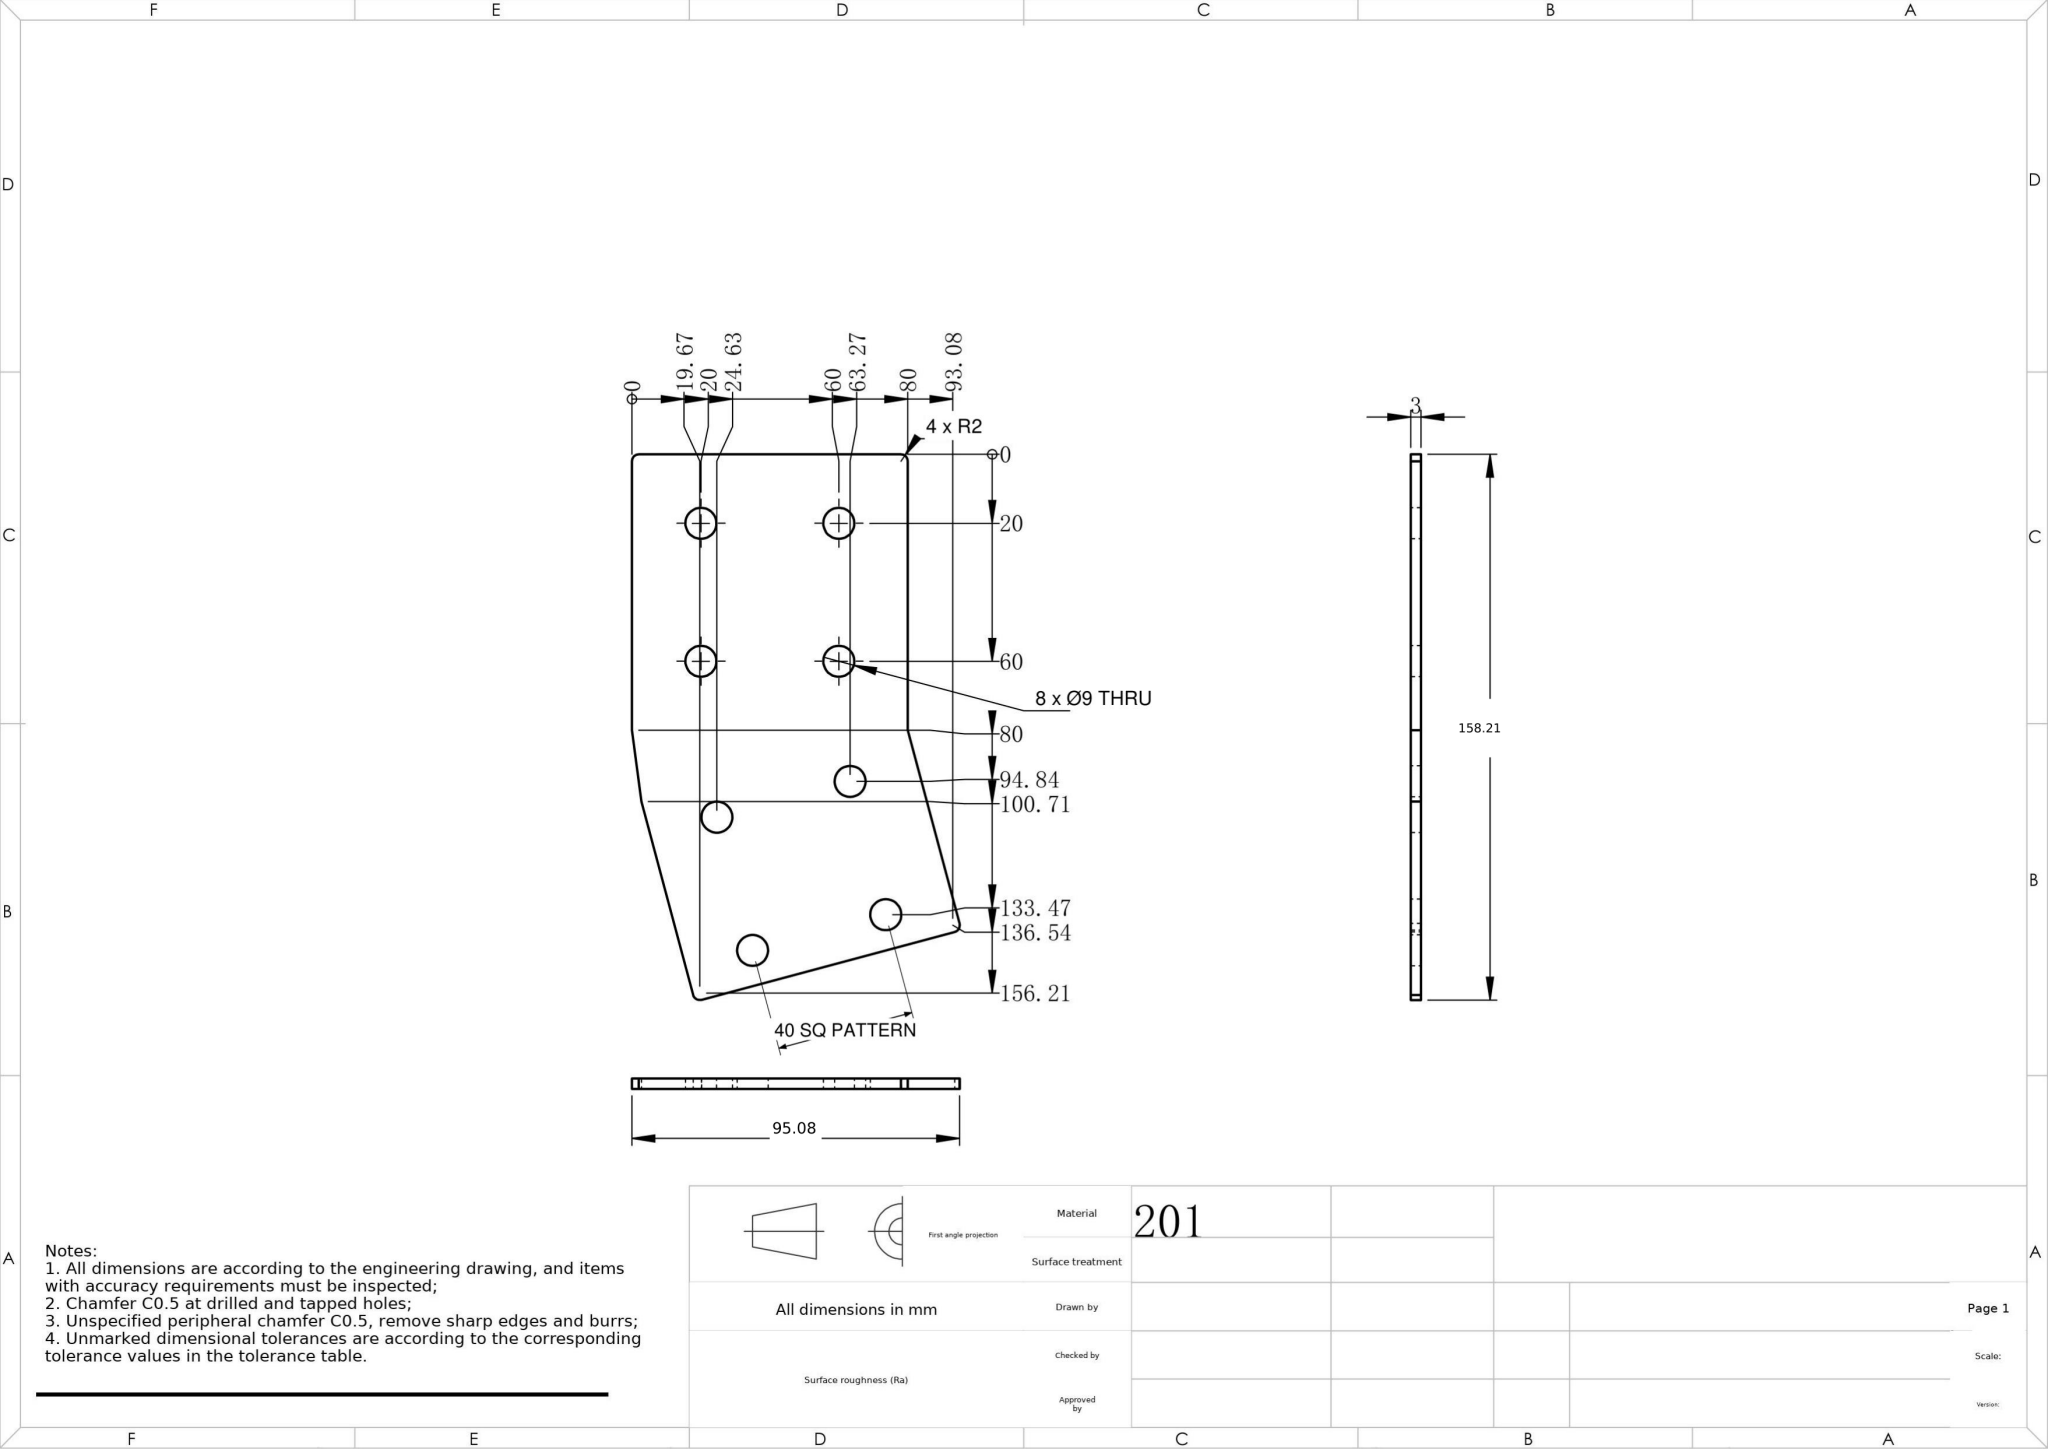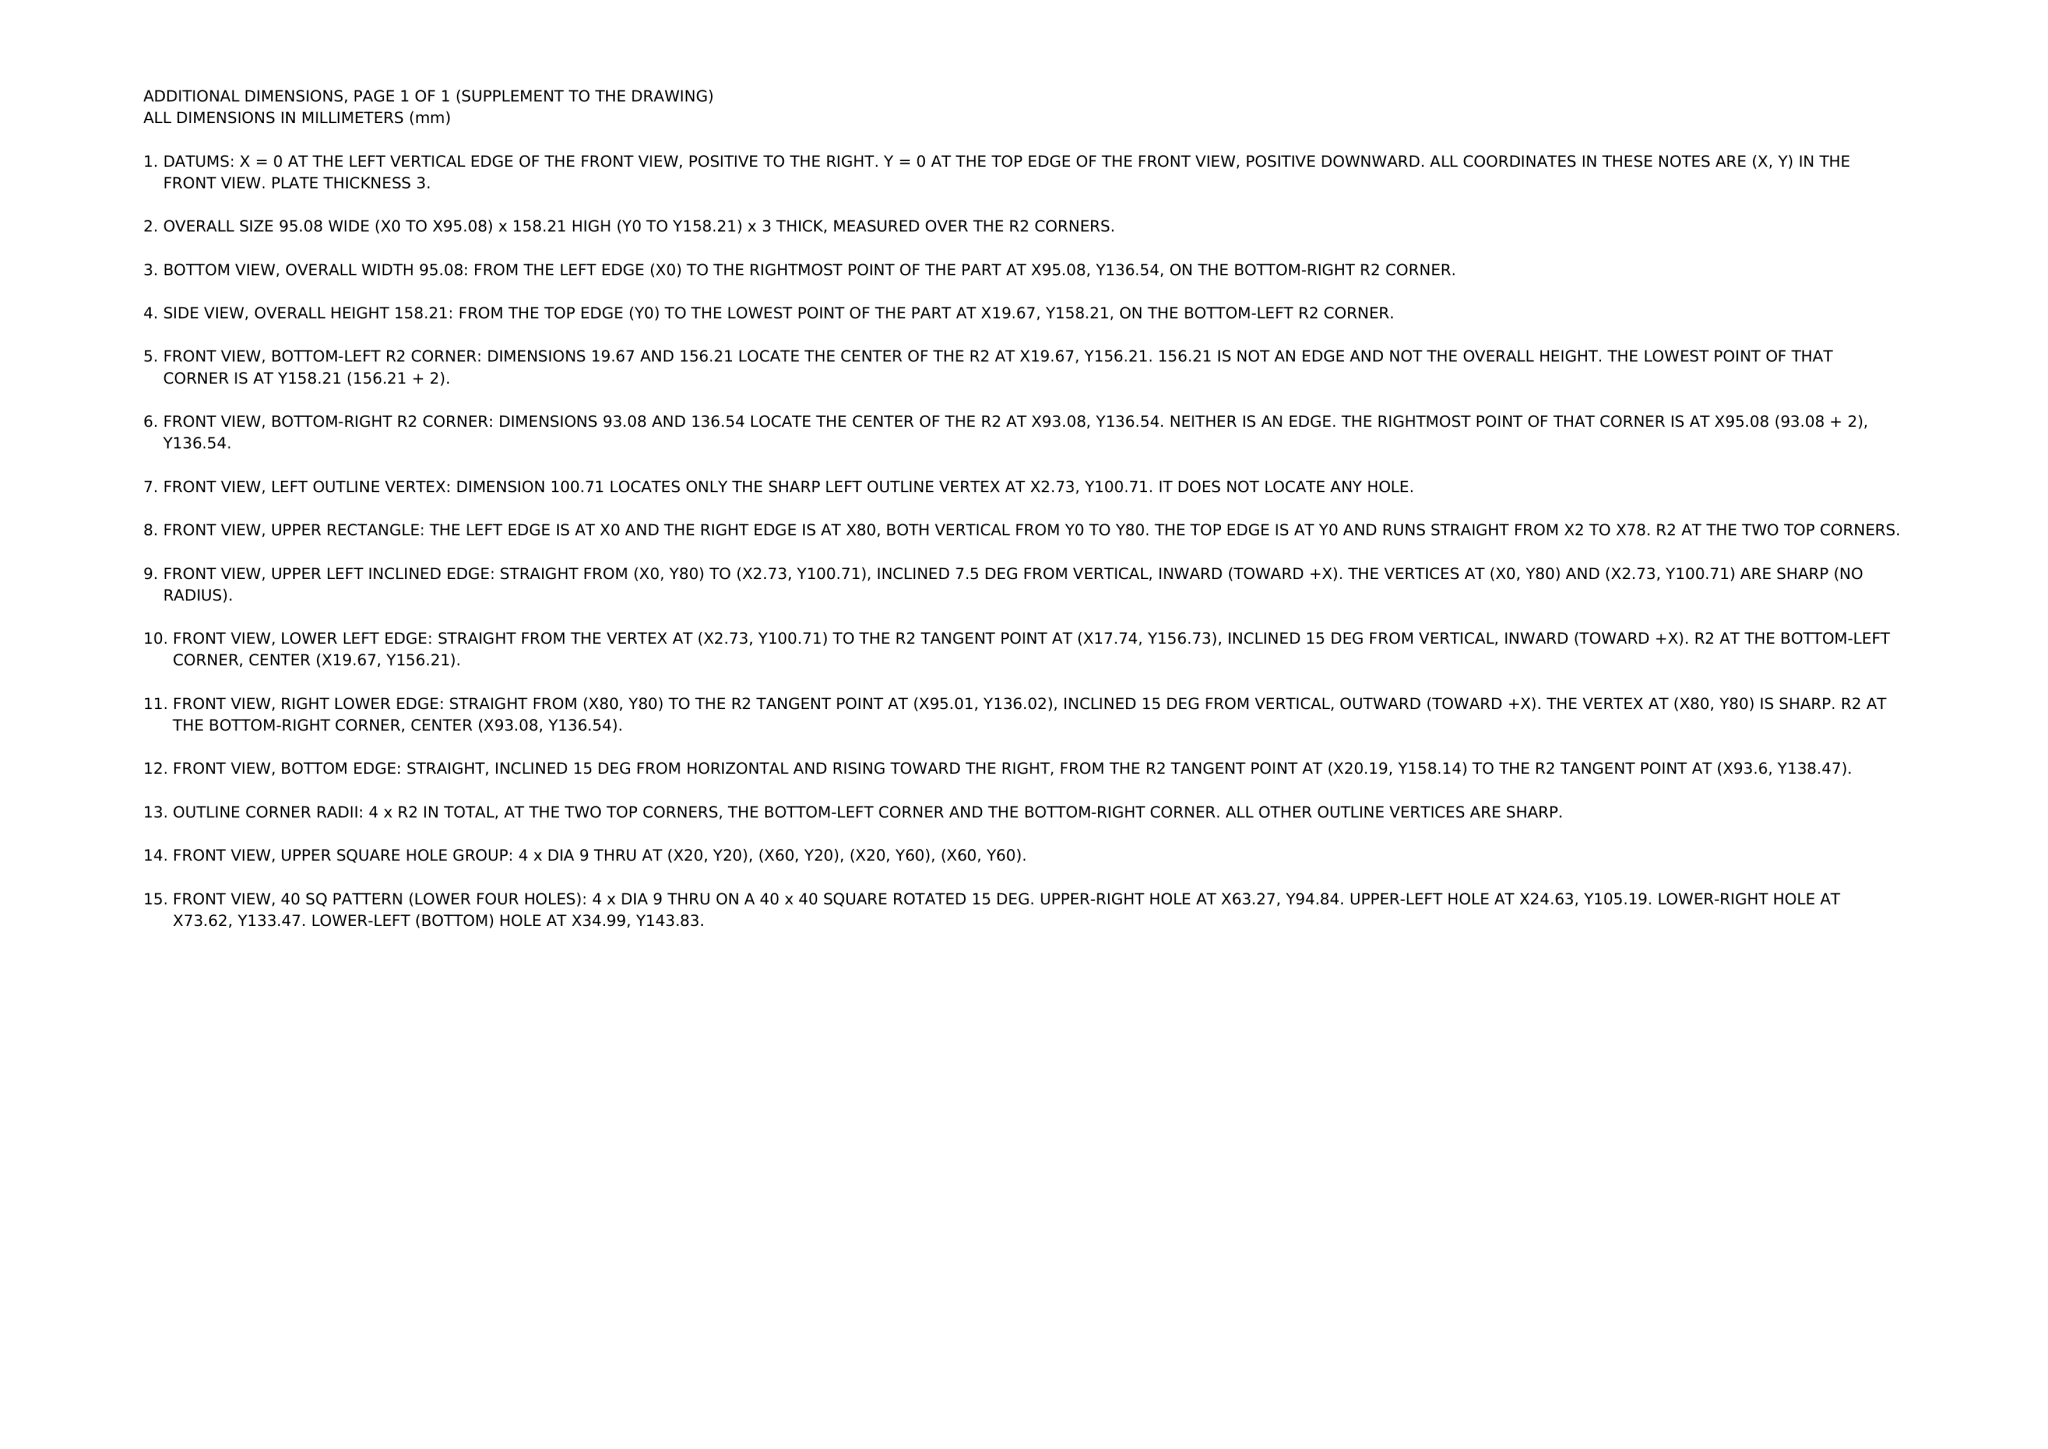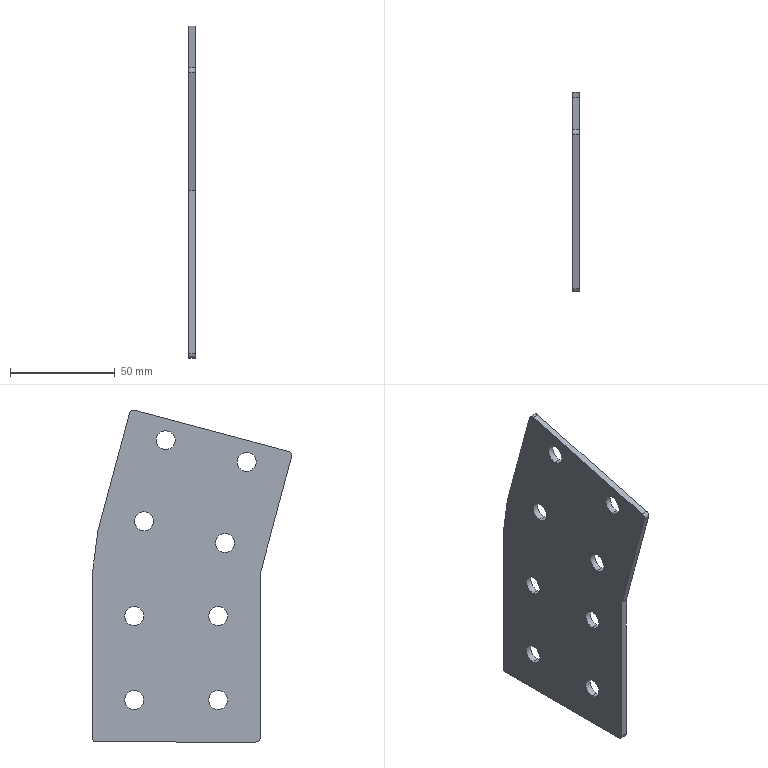Part | NX | mm | 1 solid | 29 faces | box 3 x 95.08 x 158.21 mm | volume 34548 mm3 | cylinder 20 | plane 9 | commonest cylinder face diameters 9 x16 4 x4